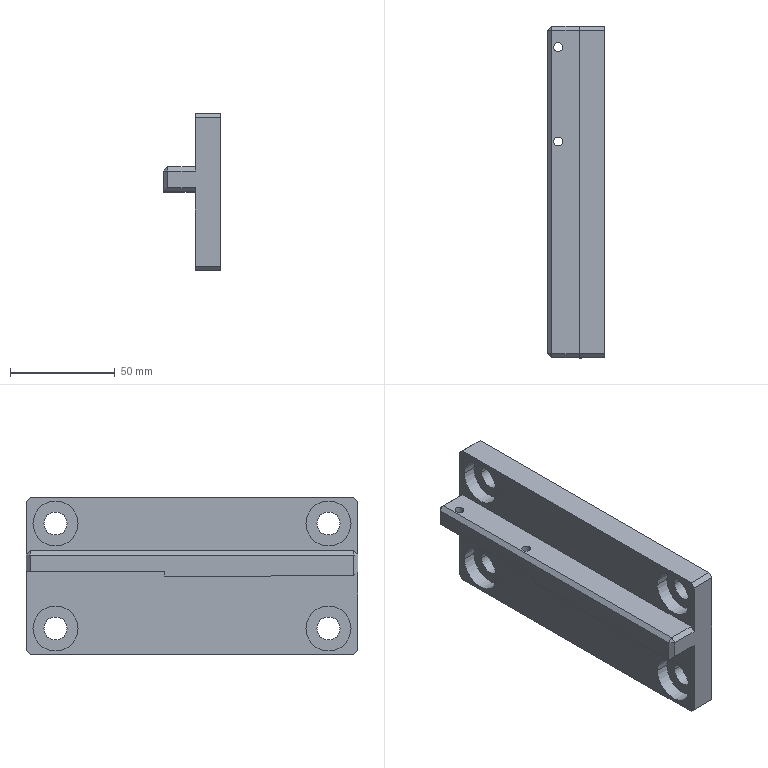Component | SolidWorks | ToolHolder-1 | 1 solid | 48 faces | box 27 x 158 x 75 mm | volume 156267 mm3 | plane 28 | cylinder 20 | commonest cylinder face diameters 21.475 x8 11 x8 4.2 x4
build123d program:
from build123d import *

# Parameters (mm, degrees)
SKETCH1_2_W                              = 158
SKETCH1_2_H                              = 75
BOSS_EXTRUDE1_DEPTH                      = 12
BOSS_EXTRUDE2_DEPTH                      = 15
M5_TAPPED_HOLE1_D                        = 4.2
CHAMFER1_SIZE                            = 2
M10_HEX_HEAD_BOLT_POST_HOLE1_D           = 11
M10_HEX_HEAD_BOLT_POST_HOLE1_CBORE_D     = 21.475
M10_HEX_HEAD_BOLT_POST_HOLE1_CBORE_DEPTH = 6.4
CHAMFER2_SIZE                            = 2
SKETCH1_W                                = 1.466
SKETCH1_H                                = 2.7
RELIEF_BLADESEAT_DEPTH                   = 15


with BuildPart() as part:
    # Sketch1_2 → Boss-Extrude1 (new body)
    with BuildSketch(Plane.XY):
        Rectangle(SKETCH1_2_W, SKETCH1_2_H)
    extrude(amount=BOSS_EXTRUDE1_DEPTH)

    # Sketch2 → Boss-Extrude2 (add)
    with BuildSketch(Plane.XY.offset(12)):
        Polygon((-79, 0), (-79, -12), (79, -12), (79, -2.2), (14, -2.2), (14, 0), align=None)
    extrude(amount=BOSS_EXTRUDE2_DEPTH)

    # M5 Tapped Hole1 (through all)
    with Locations(Plane(origin=(0, -2.2, 0), x_dir=(1, 0, 0), z_dir=(0, 1, 0))):
        with Locations((69, -22), (24, -22)):
            Hole(M5_TAPPED_HOLE1_D / 2)

    # Chamfer1
    chamfer1_edges = [part.edges().sort_by_distance(p)[0] for p in [
        (-79, 0, 19.5),
        (-79, -12, 19.5),
        (79, -12, 19.5),
        (-79, -6, 27),
        (0, -12, 27),
        (79, -7.1, 27),
    ]]
    chamfer(chamfer1_edges, length=CHAMFER1_SIZE)

    # M10 Hex Head Bolt Post Hole1 (through all)
    with Locations(Plane.XY.offset(12)):
        with Locations((65, -25), (65, 25), (-65, 25), (-65, -25)):
            CounterBoreHole(M10_HEX_HEAD_BOLT_POST_HOLE1_D / 2, M10_HEX_HEAD_BOLT_POST_HOLE1_CBORE_D / 2, M10_HEX_HEAD_BOLT_POST_HOLE1_CBORE_DEPTH)

    # Chamfer2
    chamfer2_edges = [part.edges().sort_by_distance(p)[0] for p in [
        (-79, 37.5, 6),
        (79, 37.5, 6),
        (79, -37.5, 6),
        (-79, -37.5, 6),
    ]]
    chamfer(chamfer2_edges, length=CHAMFER2_SIZE)

    # Sketch1 → Relief_BladeSeat (cut)
    with BuildSketch(Plane.XY.offset(27)):
        with Locations((14.033, -0.85)):
            Rectangle(SKETCH1_W, SKETCH1_H)
    extrude(amount=-RELIEF_BLADESEAT_DEPTH, mode=Mode.SUBTRACT)


solid = part.part

# Placed as in the assembly
solid = solid.moved(Location((-392.772, -327.766, 894.5), (-90, -90, 0)))